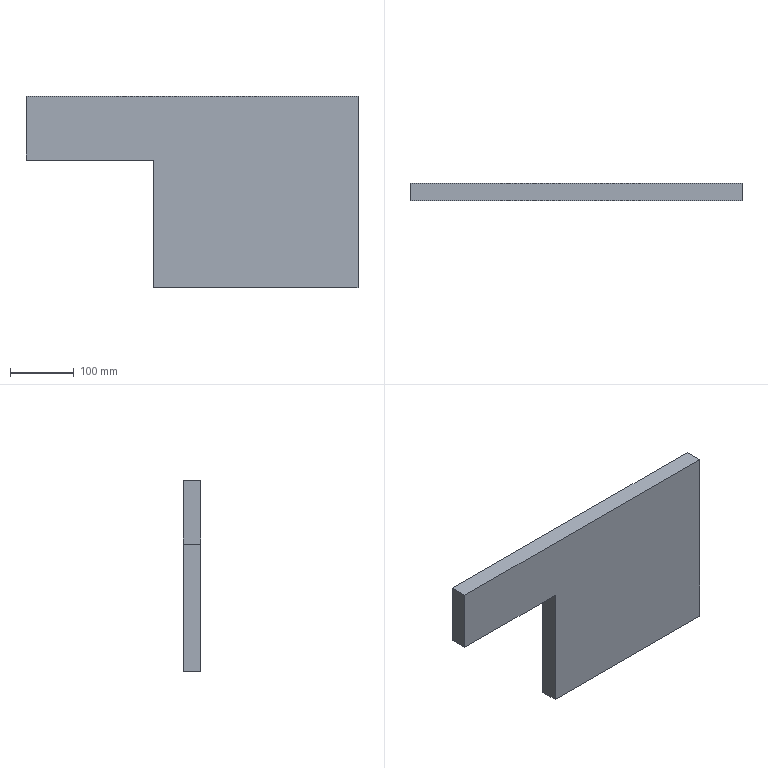Component | SolidWorks | HZ022-A001-E002-1 | 1 solid | 8 faces | box 520 x 27.5 x 300 mm | volume 3190000 mm3 | plane 8 | material AL6061
build123d program:
from build123d import *

# Parameters (mm, degrees)
SKETCH1_W           = 520
SKETCH1_H           = 300
BOSS_EXTRUDE1_DEPTH = 27.5
SKETCH2_W           = 200
SKETCH2_H           = 200
CUT_EXTRUDE1_DEPTH  = 302.424


with BuildPart() as part:
    # Sketch1 → Boss-Extrude1 (new body)
    with BuildSketch(Plane(origin=(0, 0, 0), x_dir=(1, 0, 0), z_dir=(0, 1, 0))):
        Rectangle(SKETCH1_W, SKETCH1_H)
    extrude(amount=BOSS_EXTRUDE1_DEPTH)

    # Sketch2 → Cut-Extrude1 (cut, through all)
    with BuildSketch(Plane(origin=(0, 27.5, 0), x_dir=(1, 0, 0), z_dir=(0, 1, 0))):
        with Locations((-160, 50)):
            Rectangle(SKETCH2_W, SKETCH2_H)
    extrude(amount=-CUT_EXTRUDE1_DEPTH, mode=Mode.SUBTRACT)


solid = part.part

# Placed as in the assembly
solid = solid.moved(Location((-34.556, -12.848, 800), (0, 0, 0)))
STEP:
#1=COLOUR_RGB('',0.7922,0.8196,0.9333);
#2=FILL_AREA_STYLE_COLOUR('',#1);
#3=FILL_AREA_STYLE('',(#2));
#4=SURFACE_STYLE_FILL_AREA(#3);
#5=SURFACE_SIDE_STYLE('',(#4));
#6=SURFACE_STYLE_USAGE(.BOTH.,#5);
#7=PRESENTATION_STYLE_ASSIGNMENT((#6));
#8=CARTESIAN_POINT('',(8.876,-0.5058,37.402));
#9=VERTEX_POINT('',#8);
#10=CARTESIAN_POINT('',(8.876,-0.5058,25.591));
#11=VERTEX_POINT('',#10);
#12=CARTESIAN_POINT('',(8.876,-0.5058,25.591));
#13=DIRECTION('',(0.,0.,-1.));
#14=VECTOR('',#13,39.37);
#15=LINE('',#12,#14);
#16=EDGE_CURVE('',#9,#11,#15,.T.);
#17=ORIENTED_EDGE('',*,*,#16,.T.);
#18=CARTESIAN_POINT('',(8.876,0.5769,25.591));
#19=VERTEX_POINT('',#18);
#20=CARTESIAN_POINT('',(8.876,0.5769,25.591));
#21=DIRECTION('',(0.,-1.,0.));
#22=VECTOR('',#21,39.37);
#23=LINE('',#20,#22);
#24=EDGE_CURVE('',#19,#11,#23,.T.);
#25=ORIENTED_EDGE('',*,*,#24,.F.);
#26=CARTESIAN_POINT('',(8.876,0.5769,37.402));
#27=VERTEX_POINT('',#26);
#28=CARTESIAN_POINT('',(8.876,0.5769,25.591));
#29=DIRECTION('',(0.,0.,-1.));
#30=VECTOR('',#29,39.37);
#31=LINE('',#28,#30);
#32=EDGE_CURVE('',#27,#19,#31,.T.);
#33=ORIENTED_EDGE('',*,*,#32,.F.);
#34=CARTESIAN_POINT('',(8.876,0.5769,37.402));
#35=DIRECTION('',(0.,-1.,0.));
#36=VECTOR('',#35,39.37);
#37=LINE('',#34,#36);
#38=EDGE_CURVE('',#27,#9,#37,.T.);
#39=ORIENTED_EDGE('',*,*,#38,.T.);
#40=EDGE_LOOP('',(#17,#25,#33,#39));
#41=FACE_OUTER_BOUND('',#40,.T.);
#42=CARTESIAN_POINT('',(8.876,0.5769,25.591));
#43=DIRECTION('',(-1.,0.,0.));
#44=DIRECTION('',(0.,0.,1.));
#45=AXIS2_PLACEMENT_3D('',#42,#43,#44);
#46=PLANE('',#45);
#47=ADVANCED_FACE('',(#41),#46,.F.);
#48=CARTESIAN_POINT('',(-3.723,-0.5058,25.591));
#49=VERTEX_POINT('',#48);
#50=CARTESIAN_POINT('',(-11.597,-0.5058,25.591));
#51=DIRECTION('',(-1.,0.,0.));
#52=VECTOR('',#51,39.37);
#53=LINE('',#50,#52);
#54=EDGE_CURVE('',#11,#49,#53,.T.);
#55=ORIENTED_EDGE('',*,*,#54,.T.);
#56=CARTESIAN_POINT('',(-3.723,0.5769,25.591));
#57=VERTEX_POINT('',#56);
#58=CARTESIAN_POINT('',(-3.723,-0.5058,25.591));
#59=DIRECTION('',(0.,1.,0.));
#60=VECTOR('',#59,39.37);
#61=LINE('',#58,#60);
#62=EDGE_CURVE('',#49,#57,#61,.T.);
#63=ORIENTED_EDGE('',*,*,#62,.T.);
#64=CARTESIAN_POINT('',(-11.597,0.5769,25.591));
#65=DIRECTION('',(-1.,0.,0.));
#66=VECTOR('',#65,39.37);
#67=LINE('',#64,#66);
#68=EDGE_CURVE('',#19,#57,#67,.T.);
#69=ORIENTED_EDGE('',*,*,#68,.F.);
#70=ORIENTED_EDGE('',*,*,#24,.T.);
#71=EDGE_LOOP('',(#55,#63,#69,#70));
#72=FACE_OUTER_BOUND('',#71,.T.);
#73=CARTESIAN_POINT('',(-11.597,0.5769,25.591));
#74=DIRECTION('',(0.,0.,1.));
#75=DIRECTION('',(1.,0.,0.));
#76=AXIS2_PLACEMENT_3D('',#73,#74,#75);
#77=PLANE('',#76);
#78=ADVANCED_FACE('',(#72),#77,.F.);
#79=CARTESIAN_POINT('',(-11.597,0.5769,33.465));
#80=VERTEX_POINT('',#79);
#81=CARTESIAN_POINT('',(-11.597,0.5769,37.402));
#82=VERTEX_POINT('',#81);
#83=CARTESIAN_POINT('',(-11.597,0.5769,25.591));
#84=DIRECTION('',(0.,0.,1.));
#85=VECTOR('',#84,39.37);
#86=LINE('',#83,#85);
#87=EDGE_CURVE('',#80,#82,#86,.T.);
#88=ORIENTED_EDGE('',*,*,#87,.F.);
#89=CARTESIAN_POINT('',(-11.597,-0.5058,33.465));
#90=VERTEX_POINT('',#89);
#91=CARTESIAN_POINT('',(-11.597,-0.5058,33.465));
#92=DIRECTION('',(0.,1.,0.));
#93=VECTOR('',#92,39.37);
#94=LINE('',#91,#93);
#95=EDGE_CURVE('',#90,#80,#94,.T.);
#96=ORIENTED_EDGE('',*,*,#95,.F.);
#97=CARTESIAN_POINT('',(-11.597,-0.5058,37.402));
#98=VERTEX_POINT('',#97);
#99=CARTESIAN_POINT('',(-11.597,-0.5058,25.591));
#100=DIRECTION('',(0.,0.,1.));
#101=VECTOR('',#100,39.37);
#102=LINE('',#99,#101);
#103=EDGE_CURVE('',#90,#98,#102,.T.);
#104=ORIENTED_EDGE('',*,*,#103,.T.);
#105=CARTESIAN_POINT('',(-11.597,0.5769,37.402));
#106=DIRECTION('',(0.,-1.,0.));
#107=VECTOR('',#106,39.37);
#108=LINE('',#105,#107);
#109=EDGE_CURVE('',#82,#98,#108,.T.);
#110=ORIENTED_EDGE('',*,*,#109,.F.);
#111=EDGE_LOOP('',(#88,#96,#104,#110));
#112=FACE_OUTER_BOUND('',#111,.T.);
#113=CARTESIAN_POINT('',(-11.597,0.5769,25.591));
#114=DIRECTION('',(1.,0.,-0.));
#115=DIRECTION('',(-0.,0.,-1.));
#116=AXIS2_PLACEMENT_3D('',#113,#114,#115);
#117=PLANE('',#116);
#118=ADVANCED_FACE('',(#112),#117,.F.);
#119=CARTESIAN_POINT('',(-11.597,-0.5058,37.402));
#120=DIRECTION('',(1.,0.,0.));
#121=VECTOR('',#120,39.37);
#122=LINE('',#119,#121);
#123=EDGE_CURVE('',#98,#9,#122,.T.);
#124=ORIENTED_EDGE('',*,*,#123,.T.);
#125=ORIENTED_EDGE('',*,*,#38,.F.);
#126=CARTESIAN_POINT('',(-11.597,0.5769,37.402));
#127=DIRECTION('',(1.,0.,0.));
#128=VECTOR('',#127,39.37);
#129=LINE('',#126,#128);
#130=EDGE_CURVE('',#82,#27,#129,.T.);
#131=ORIENTED_EDGE('',*,*,#130,.F.);
#132=ORIENTED_EDGE('',*,*,#109,.T.);
#133=EDGE_LOOP('',(#124,#125,#131,#132));
#134=FACE_OUTER_BOUND('',#133,.T.);
#135=CARTESIAN_POINT('',(-11.597,0.5769,37.402));
#136=DIRECTION('',(0.,0.,-1.));
#137=DIRECTION('',(-1.,0.,0.));
#138=AXIS2_PLACEMENT_3D('',#135,#136,#137);
#139=PLANE('',#138);
#140=ADVANCED_FACE('',(#134),#139,.F.);
#141=CARTESIAN_POINT('',(-3.723,0.5769,33.465));
#142=VERTEX_POINT('',#141);
#143=CARTESIAN_POINT('',(-3.723,0.5769,25.591));
#144=DIRECTION('',(-0.,0.,-1.));
#145=VECTOR('',#144,39.37);
#146=LINE('',#143,#145);
#147=EDGE_CURVE('',#142,#57,#146,.T.);
#148=ORIENTED_EDGE('',*,*,#147,.F.);
#149=CARTESIAN_POINT('',(-11.597,0.5769,33.465));
#150=DIRECTION('',(1.,0.,0.));
#151=VECTOR('',#150,39.37);
#152=LINE('',#149,#151);
#153=EDGE_CURVE('',#80,#142,#152,.T.);
#154=ORIENTED_EDGE('',*,*,#153,.F.);
#155=ORIENTED_EDGE('',*,*,#87,.T.);
#156=ORIENTED_EDGE('',*,*,#130,.T.);
#157=ORIENTED_EDGE('',*,*,#32,.T.);
#158=ORIENTED_EDGE('',*,*,#68,.T.);
#159=EDGE_LOOP('',(#148,#154,#155,#156,#157,#158));
#160=FACE_OUTER_BOUND('',#159,.T.);
#161=CARTESIAN_POINT('',(-1.36,0.5769,31.496));
#162=DIRECTION('',(0.,1.,0.));
#163=DIRECTION('',(0.,0.,1.));
#164=AXIS2_PLACEMENT_3D('',#161,#162,#163);
#165=PLANE('',#164);
#166=ADVANCED_FACE('',(#160),#165,.T.);
#167=CARTESIAN_POINT('',(-3.723,-0.5058,33.465));
#168=VERTEX_POINT('',#167);
#169=CARTESIAN_POINT('',(-11.597,-0.5058,33.465));
#170=DIRECTION('',(1.,0.,0.));
#171=VECTOR('',#170,39.37);
#172=LINE('',#169,#171);
#173=EDGE_CURVE('',#90,#168,#172,.T.);
#174=ORIENTED_EDGE('',*,*,#173,.T.);
#175=CARTESIAN_POINT('',(-3.723,-0.5058,25.591));
#176=DIRECTION('',(-0.,0.,-1.));
#177=VECTOR('',#176,39.37);
#178=LINE('',#175,#177);
#179=EDGE_CURVE('',#168,#49,#178,.T.);
#180=ORIENTED_EDGE('',*,*,#179,.T.);
#181=ORIENTED_EDGE('',*,*,#54,.F.);
#182=ORIENTED_EDGE('',*,*,#16,.F.);
#183=ORIENTED_EDGE('',*,*,#123,.F.);
#184=ORIENTED_EDGE('',*,*,#103,.F.);
#185=EDGE_LOOP('',(#174,#180,#181,#182,#183,#184));
#186=FACE_OUTER_BOUND('',#185,.T.);
#187=CARTESIAN_POINT('',(-1.36,-0.5058,31.496));
#188=DIRECTION('',(0.,1.,0.));
#189=DIRECTION('',(0.,0.,1.));
#190=AXIS2_PLACEMENT_3D('',#187,#188,#189);
#191=PLANE('',#190);
#192=ADVANCED_FACE('',(#186),#191,.F.);
#193=ORIENTED_EDGE('',*,*,#147,.T.);
#194=ORIENTED_EDGE('',*,*,#62,.F.);
#195=ORIENTED_EDGE('',*,*,#179,.F.);
#196=CARTESIAN_POINT('',(-3.723,-0.5058,33.465));
#197=DIRECTION('',(0.,1.,0.));
#198=VECTOR('',#197,39.37);
#199=LINE('',#196,#198);
#200=EDGE_CURVE('',#168,#142,#199,.T.);
#201=ORIENTED_EDGE('',*,*,#200,.T.);
#202=EDGE_LOOP('',(#193,#194,#195,#201));
#203=FACE_OUTER_BOUND('',#202,.T.);
#204=CARTESIAN_POINT('',(-3.723,-0.5058,25.591));
#205=DIRECTION('',(1.,0.,-0.));
#206=DIRECTION('',(-0.,0.,-1.));
#207=AXIS2_PLACEMENT_3D('',#204,#205,#206);
#208=PLANE('',#207);
#209=ADVANCED_FACE('',(#203),#208,.F.);
#210=ORIENTED_EDGE('',*,*,#153,.T.);
#211=ORIENTED_EDGE('',*,*,#200,.F.);
#212=ORIENTED_EDGE('',*,*,#173,.F.);
#213=ORIENTED_EDGE('',*,*,#95,.T.);
#214=EDGE_LOOP('',(#210,#211,#212,#213));
#215=FACE_OUTER_BOUND('',#214,.T.);
#216=CARTESIAN_POINT('',(-11.597,-0.5058,33.465));
#217=DIRECTION('',(0.,0.,1.));
#218=DIRECTION('',(1.,0.,0.));
#219=AXIS2_PLACEMENT_3D('',#216,#217,#218);
#220=PLANE('',#219);
#221=ADVANCED_FACE('',(#215),#220,.F.);
#222=CLOSED_SHELL('',(#47,#78,#118,#140,#166,#192,#209,#221));
#223=MANIFOLD_SOLID_BREP('',#222);
#224=STYLED_ITEM('',(#7),#223);
#225=PRESENTATION_LAYER_ASSIGNMENT('','',(#224));
#226=CARTESIAN_POINT('',(0.,0.,0.));
#227=DIRECTION('',(0.,0.,1.));
#228=DIRECTION('',(1.,0.,0.));
#229=AXIS2_PLACEMENT_3D('',#226,#227,#228);
#230=(LENGTH_UNIT()NAMED_UNIT(*)SI_UNIT($,.METRE.));
#231=LENGTH_MEASURE_WITH_UNIT(LENGTH_MEASURE(0.0254),#230);
#232=DIMENSIONAL_EXPONENTS(1.,0.,0.,0.,0.,0.,0.);
#233=(CONVERSION_BASED_UNIT('',#231)LENGTH_UNIT()NAMED_UNIT(#232));
#234=UNCERTAINTY_MEASURE_WITH_UNIT(LENGTH_MEASURE(0.00001),#233,'','');
#235=(NAMED_UNIT(*)PLANE_ANGLE_UNIT()SI_UNIT($,.RADIAN.));
#236=(NAMED_UNIT(*)SI_UNIT($,.STERADIAN.)SOLID_ANGLE_UNIT());
#237=(GEOMETRIC_REPRESENTATION_CONTEXT(3)GLOBAL_UNCERTAINTY_ASSIGNED_CONTEXT((#234))GLOBAL_UNIT_ASSIGNED_CONTEXT((#233,#235,#236))REPRESENTATION_CONTEXT('',''));
#238=ADVANCED_BREP_SHAPE_REPRESENTATION('',(#223,#229),#237);
#239=(LENGTH_UNIT()NAMED_UNIT(*)SI_UNIT($,.METRE.));
#240=LENGTH_MEASURE_WITH_UNIT(LENGTH_MEASURE(0.0254),#239);
#241=DIMENSIONAL_EXPONENTS(1.,0.,0.,0.,0.,0.,0.);
#242=(CONVERSION_BASED_UNIT('',#240)LENGTH_UNIT()NAMED_UNIT(#241));
#243=UNCERTAINTY_MEASURE_WITH_UNIT(LENGTH_MEASURE(0.00001),#242,'','');
#244=(NAMED_UNIT(*)PLANE_ANGLE_UNIT()SI_UNIT($,.RADIAN.));
#245=(NAMED_UNIT(*)SI_UNIT($,.STERADIAN.)SOLID_ANGLE_UNIT());
#246=(GEOMETRIC_REPRESENTATION_CONTEXT(3)GLOBAL_UNCERTAINTY_ASSIGNED_CONTEXT((#243))GLOBAL_UNIT_ASSIGNED_CONTEXT((#242,#244,#245))REPRESENTATION_CONTEXT('',''));
#247=MECHANICAL_DESIGN_GEOMETRIC_PRESENTATION_REPRESENTATION('',(#224),#246);